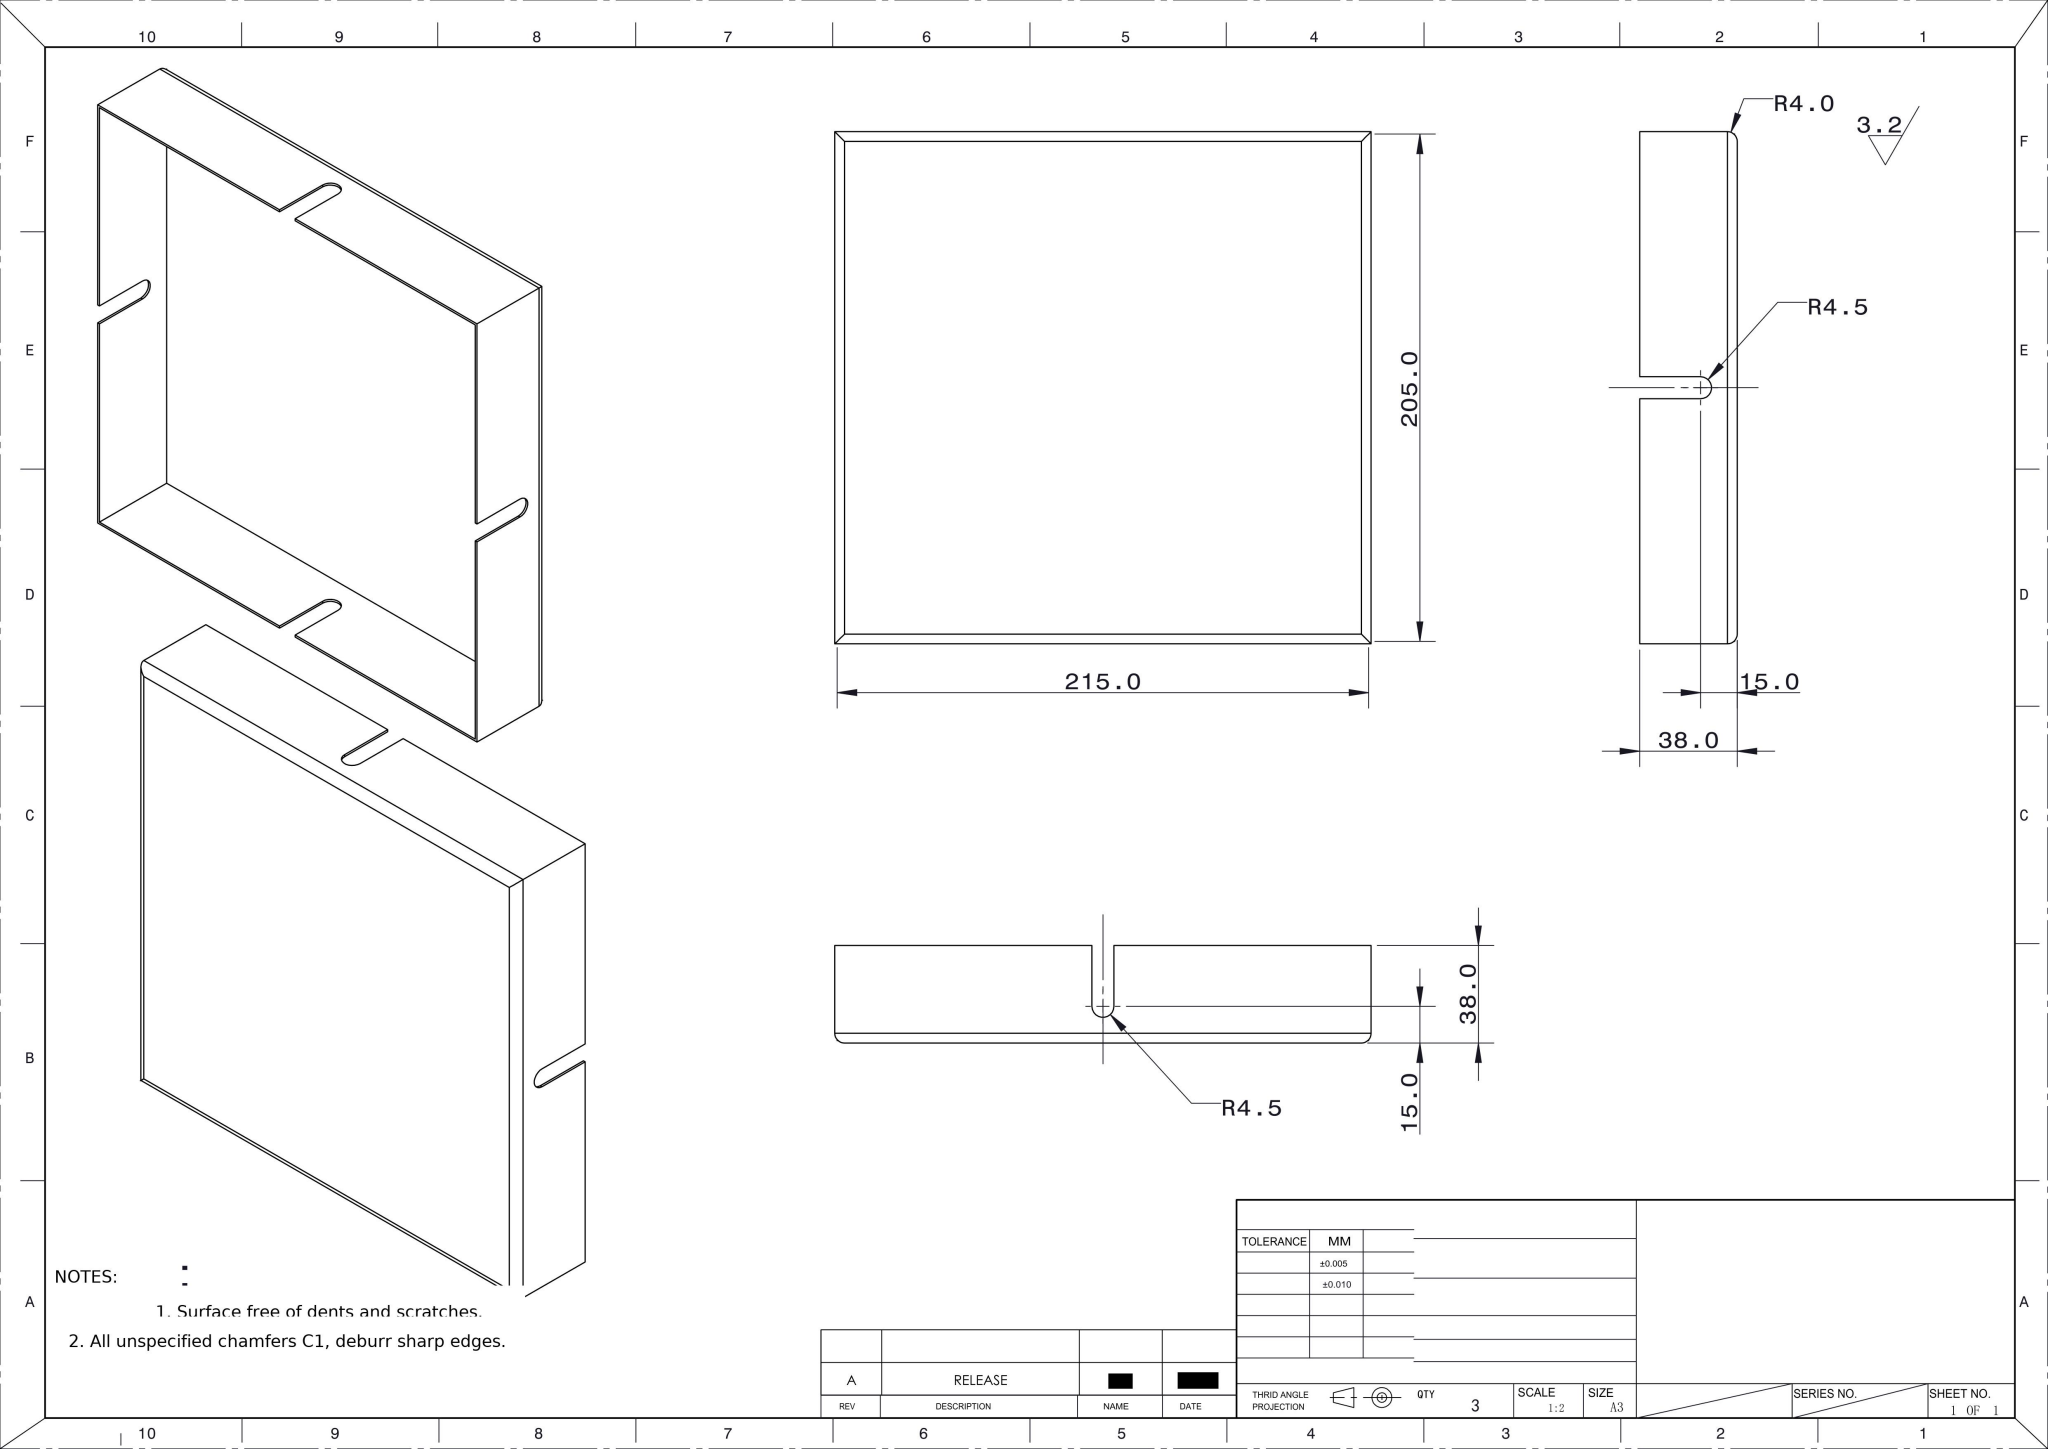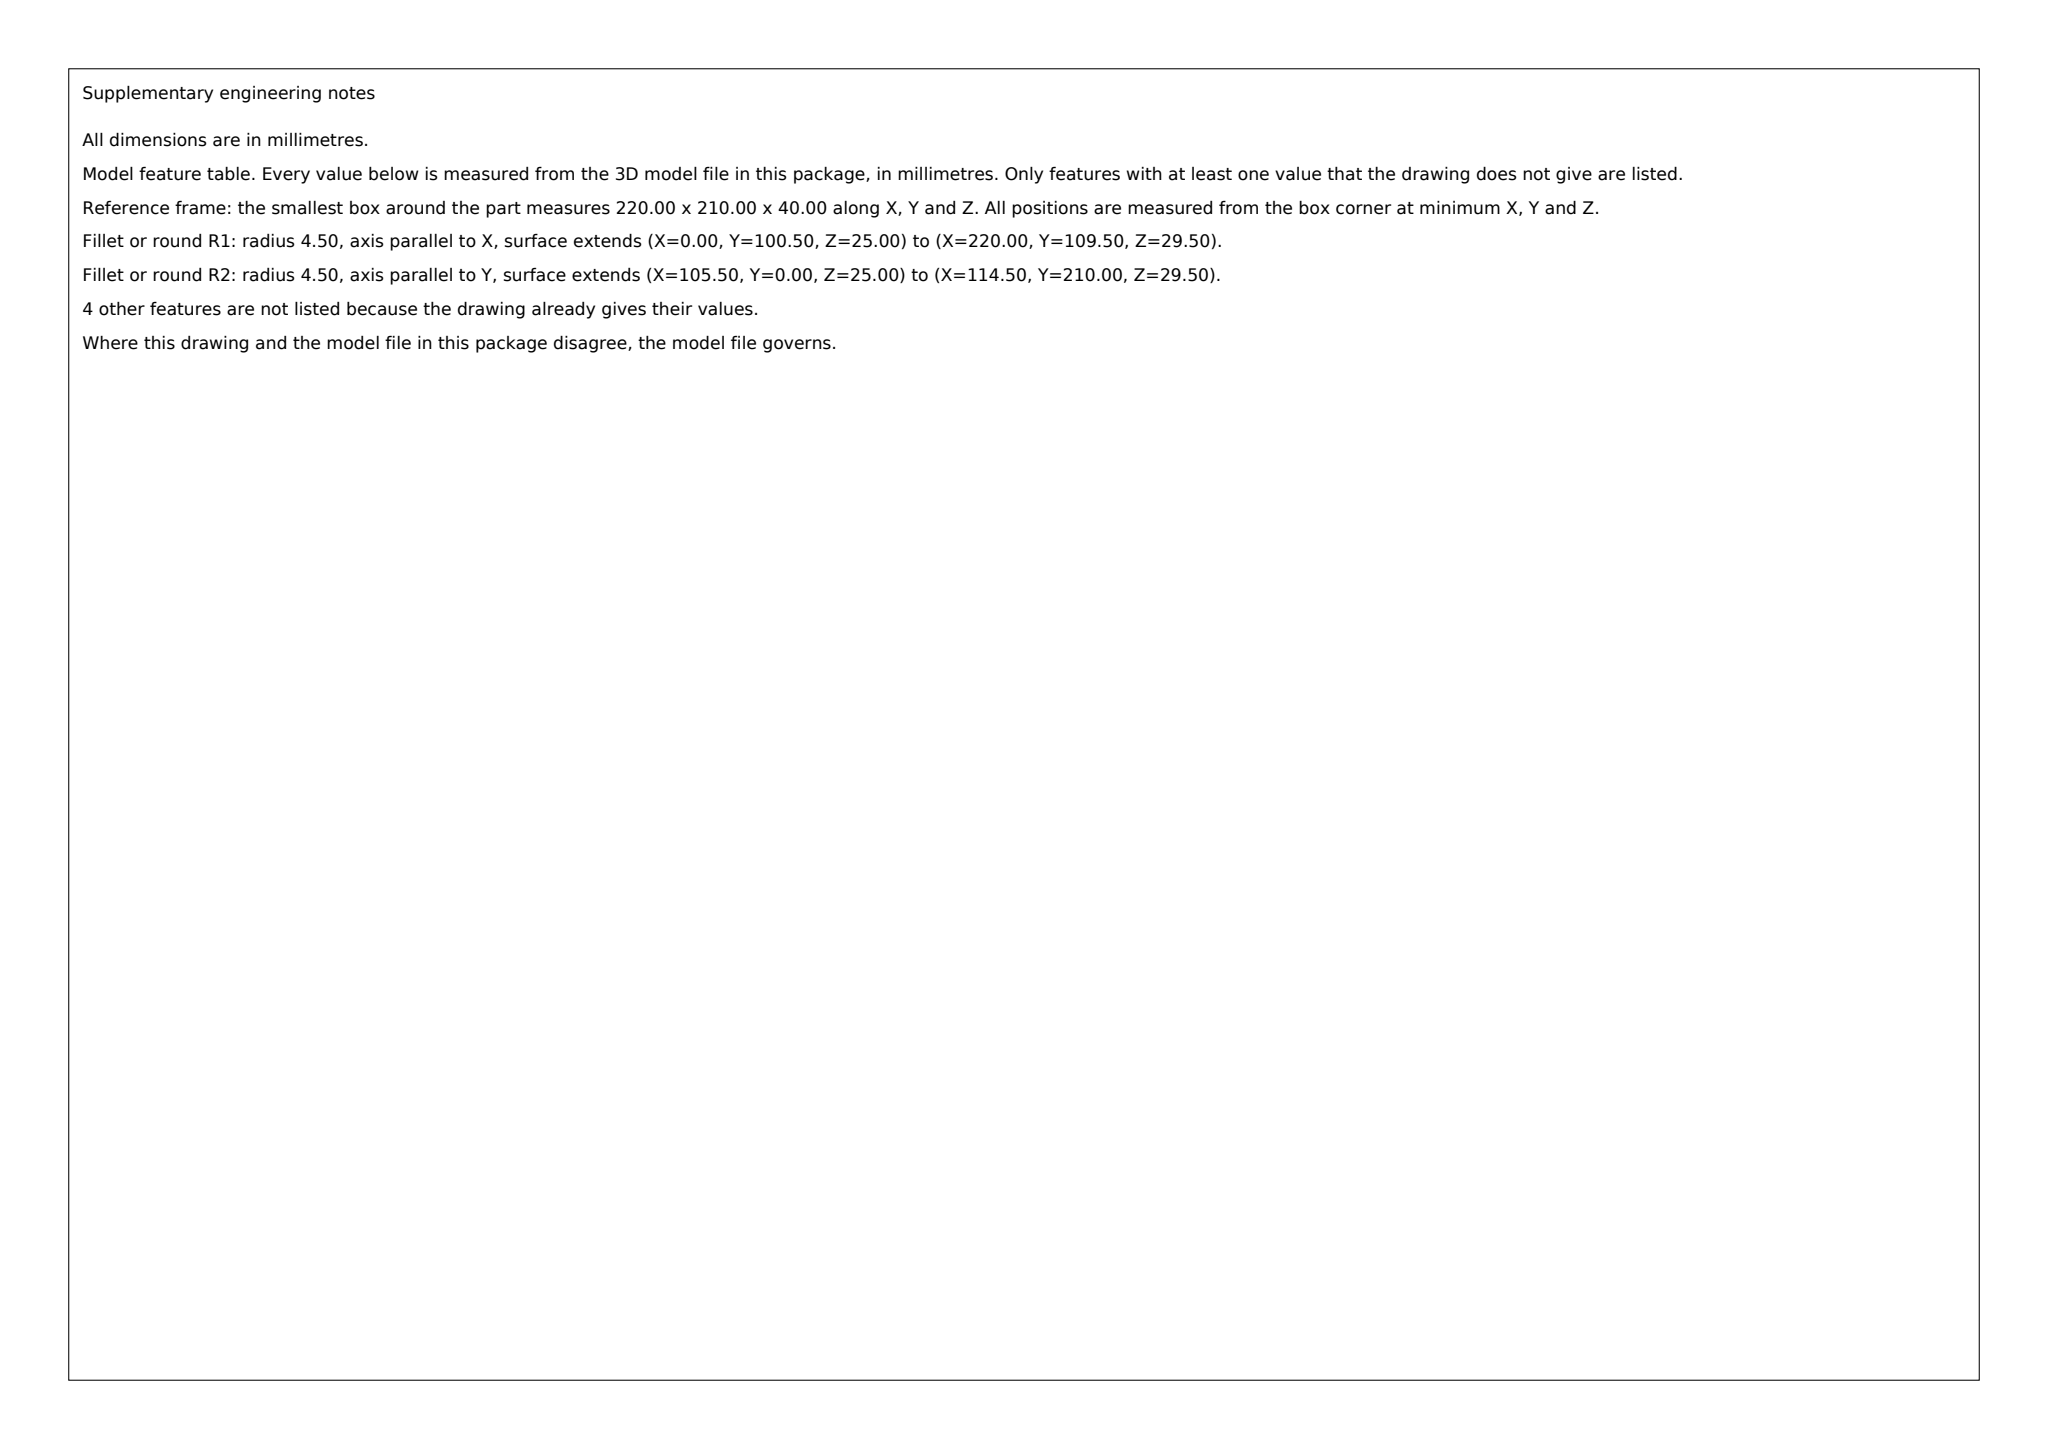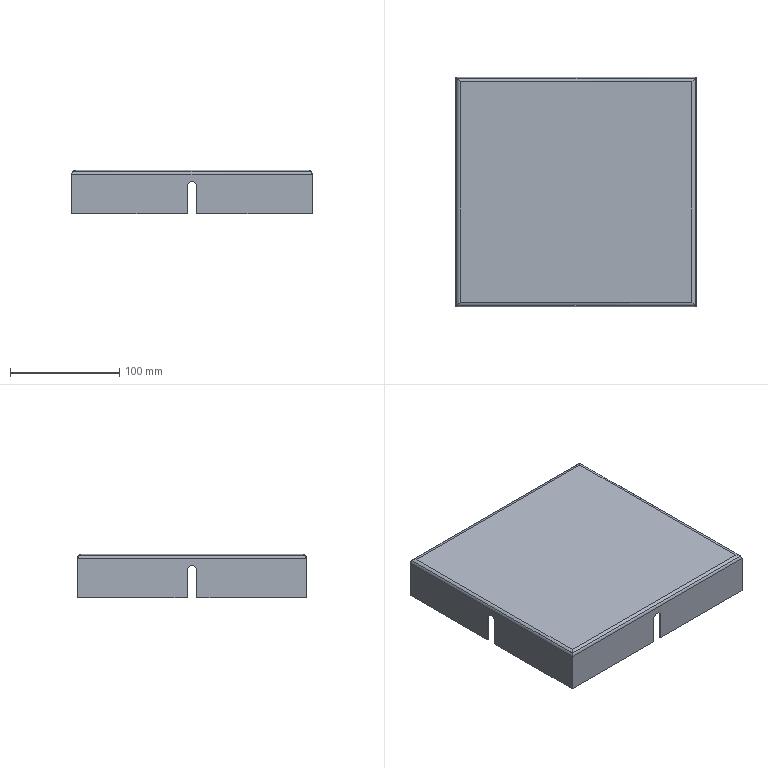Part | SolidWorks | mm | 1 solid | 30 faces | box 220 x 210 x 40 mm | volume 75628 mm3 | plane 22 | cylinder 8 | commonest cylinder face diameters 8 x4 9 x4
build123d program:
from build123d import *

# Parameters (mm, degrees)
SKETCH1_W           = 220
SKETCH1_H           = 210
BOSS_EXTRUDE1_DEPTH = 40
SHELL1_T            = -1
FILLET1_R           = 4
CUT_EXTRUDE1_DEPTH  = 260.452
CUT_EXTRUDE2_DEPTH  = 818.716


with BuildPart() as part:
    # Sketch1 → Boss-Extrude1 (new body)
    with BuildSketch(Plane.XY):
        with Locations((-37.021, 681.549)):
            Rectangle(SKETCH1_W, SKETCH1_H)
    extrude(amount=-BOSS_EXTRUDE1_DEPTH)

    # Shell1
    shell1_openings = [part.faces().sort_by_distance(p)[0] for p in [
        (-37.021, 681.549, -40),
    ]]
    offset(amount=SHELL1_T, openings=shell1_openings, kind=Kind.INTERSECTION)

    # Fillet1
    fillet1_edges = [part.edges().sort_by_distance(p)[0] for p in [
        (-37.021, 786.549, 0),
        (72.979, 681.549, 0),
        (-37.021, 576.549, 0),
        (-147.021, 681.549, 0),
    ]]
    fillet(fillet1_edges, radius=FILLET1_R)

    # Sketch3 → Cut-Extrude1 (cut, through all)
    with BuildSketch(Plane.XZ.offset(-576.549)):
        with BuildLine():
            Line((-41.521, -45), (-41.521, -15))
            ThreePointArc((-41.521, -15), (-37.021, -10.5), (-32.521, -15))
            Line((-32.521, -15), (-32.521, -45))
            ThreePointArc((-32.521, -45), (-37.021, -49.5), (-41.521, -45))
        make_face()
    extrude(amount=-CUT_EXTRUDE1_DEPTH, mode=Mode.SUBTRACT)

    # Sketch4 → Cut-Extrude2 (cut, through all)
    with BuildSketch(Plane(origin=(72.979, 0, 0), x_dir=(0, 0, -1), z_dir=(1, 0, 0))):
        with BuildLine():
            Line((15, 686.049), (45, 686.049))
            ThreePointArc((45, 686.049), (49.5, 681.549), (45, 677.049))
            Line((45, 677.049), (15, 677.049))
            ThreePointArc((15, 677.049), (10.5, 681.549), (15, 686.049))
        make_face()
    extrude(amount=-CUT_EXTRUDE2_DEPTH, mode=Mode.SUBTRACT)


solid = part.part